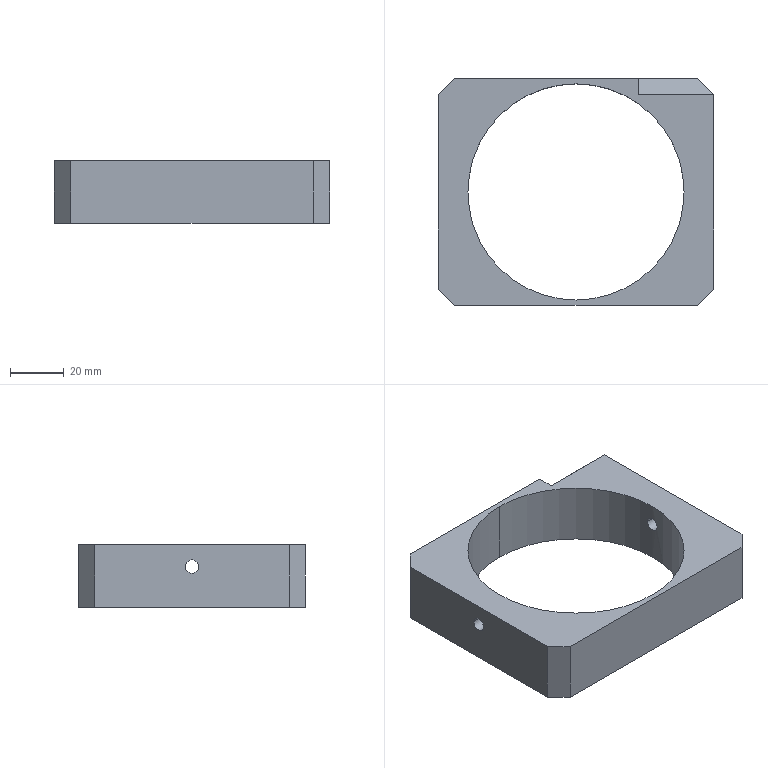CAM job | Mastercam | mm | 19 operations | part box 102 x 84 x 23
1. Facing | 13 - 50 圆鼻铣刀
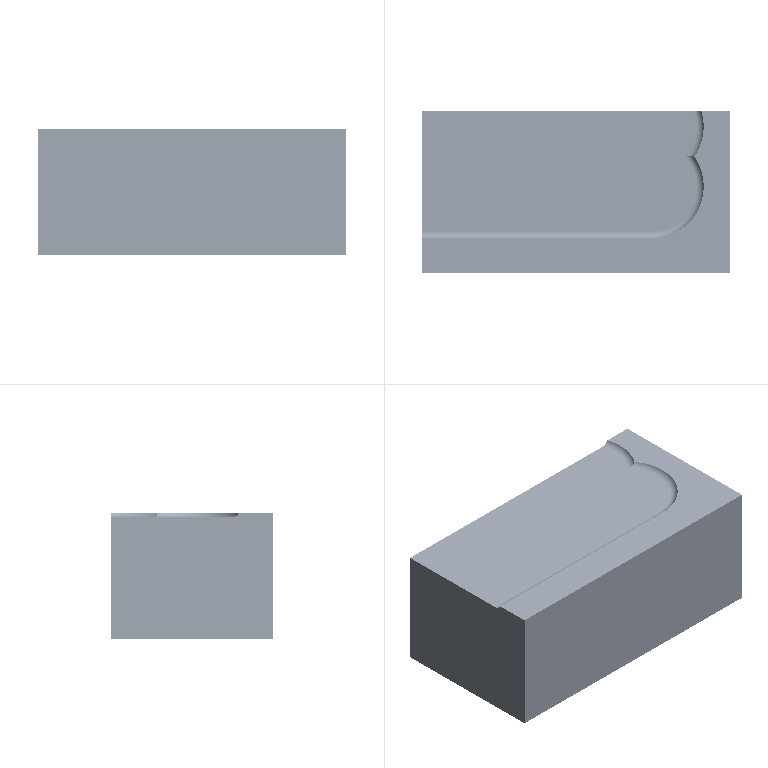2. 2D High Speed (2D Dynamic Mill) | 2 - 12 平铣刀
3. 2D High Speed (2D Dynamic Mill) | 2 - 12 平铣刀
4. Contour (2D) | 3 - 12 平铣刀
5. Contour (2D) | 3 - 12 平铣刀
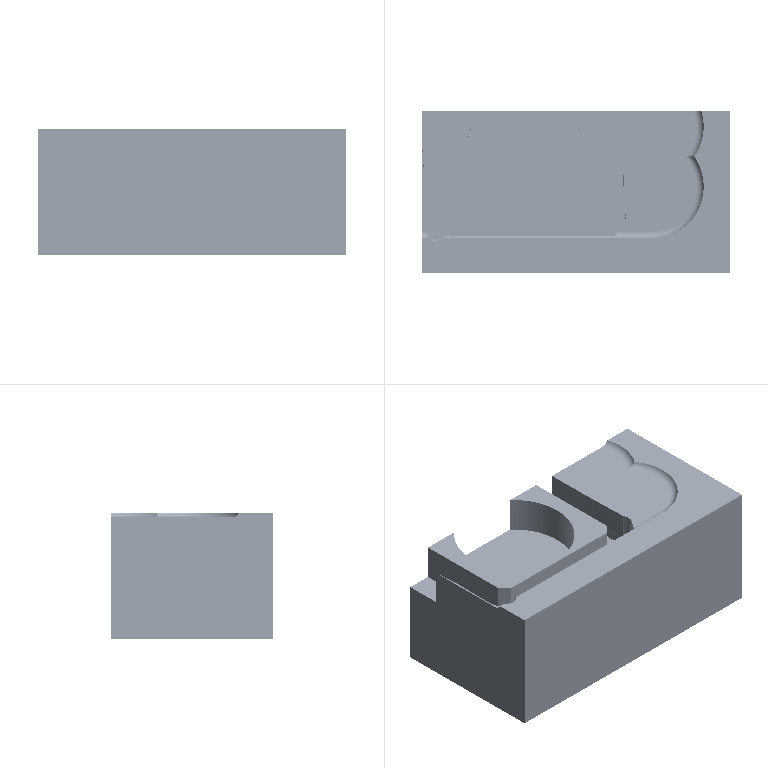6. Contour (2D chamfer) | 6 - 6 倒角刀
7. Facing | 13 - 50 圆鼻铣刀
8. Facing | 13 - 50 圆鼻铣刀
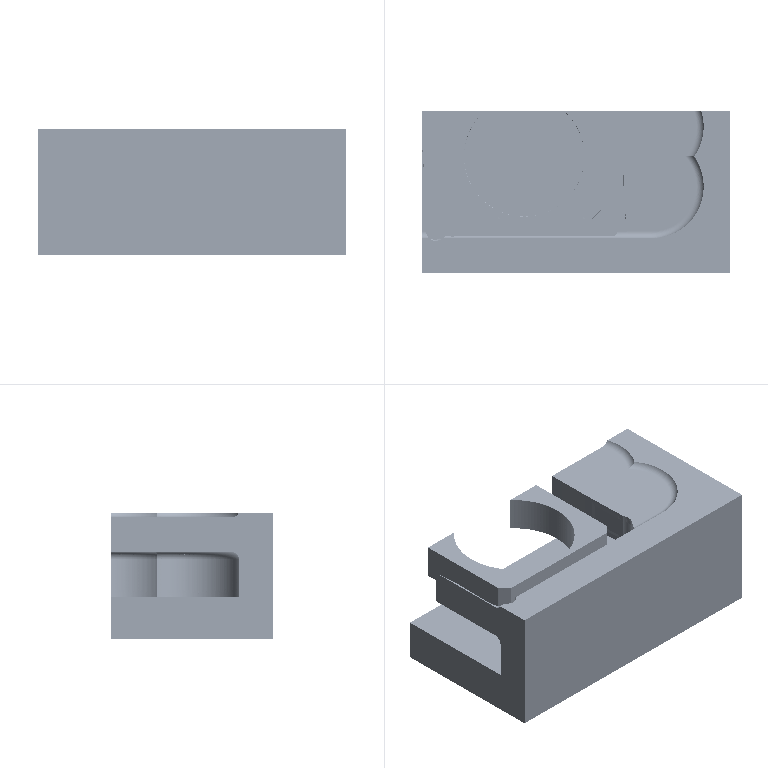9. Contour (Ramp) | 2 - 12 平铣刀
10. Contour (2D) | 3 - 12 平铣刀
11. Model Chamfer | 6 - 6 倒角刀
12. Drill/Counterbore | 6 - 6 倒角刀
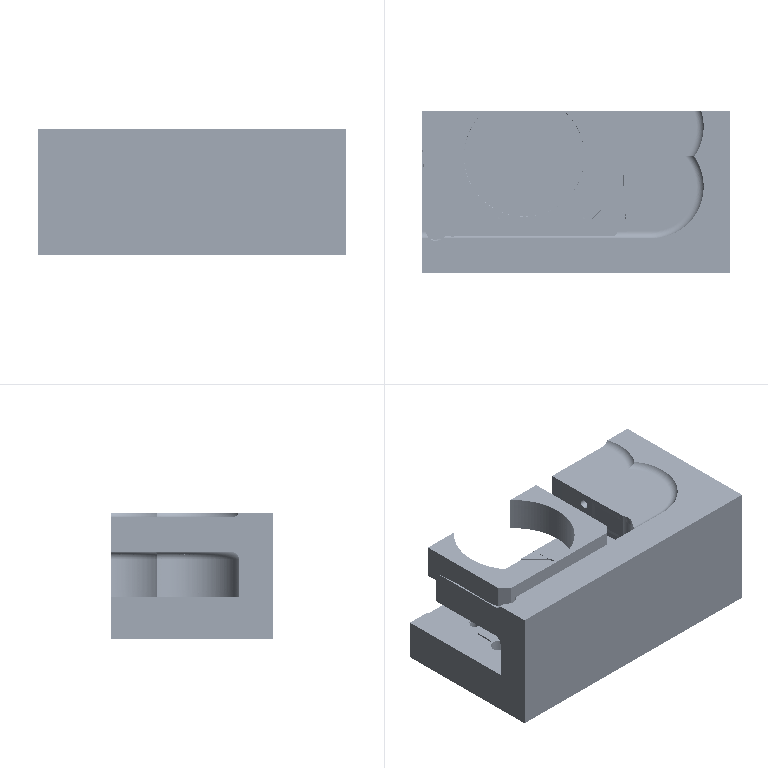13. Peck Drill | 19 - 5 钻头
14. Chamfer Drill | 6 - 6 倒角刀
15. Contour (Ramp) | 2 - 12 平铣刀
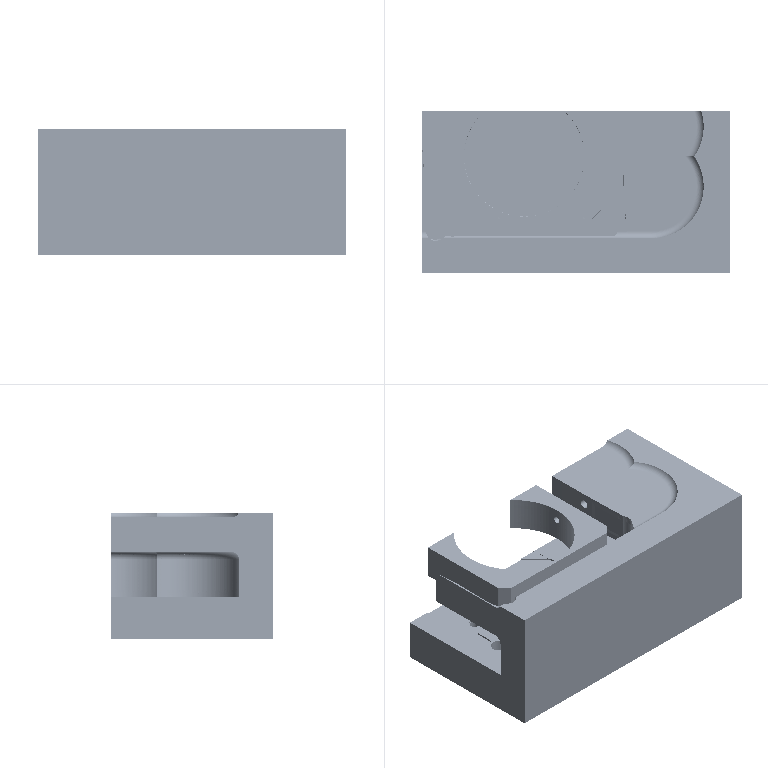16. Contour (2D) | 3 - 12 平铣刀
17. Drill/Counterbore | 6 - 6 倒角刀
18. Peck Drill | 19 - 5 钻头
19. Chamfer Drill | 6 - 6 倒角刀